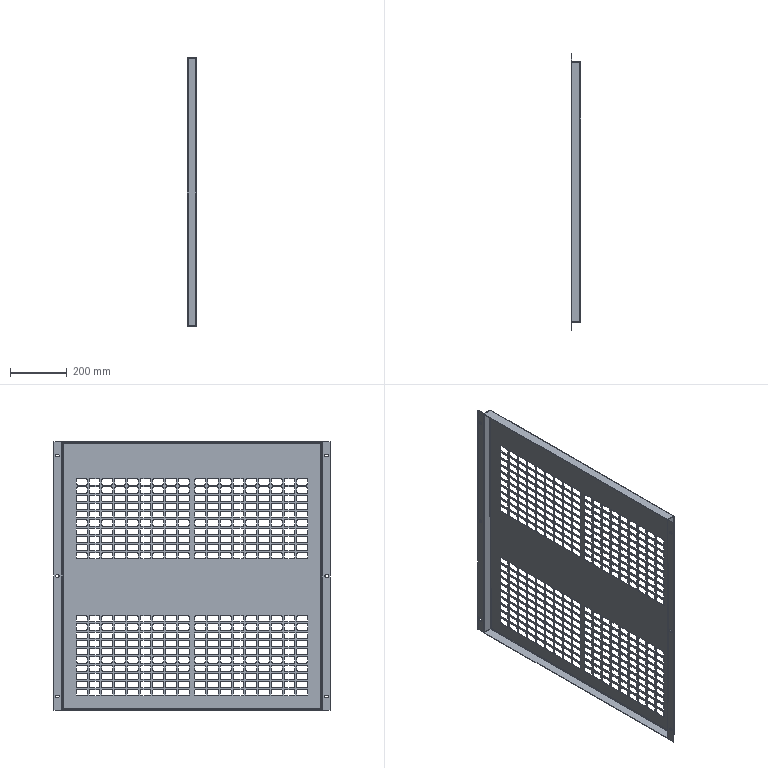Component | SolidWorks | AirInletVentAssembly-1_AirInletVent-1 | 1 solid | 2964 faces | volume 1476140 mm3 | plane 1486 | cylinder 1470 | spline 8 | commonest cylinder face diameters 6 x1440 10 x18 4 x6 8 x6 | material Plain Carbon Steel